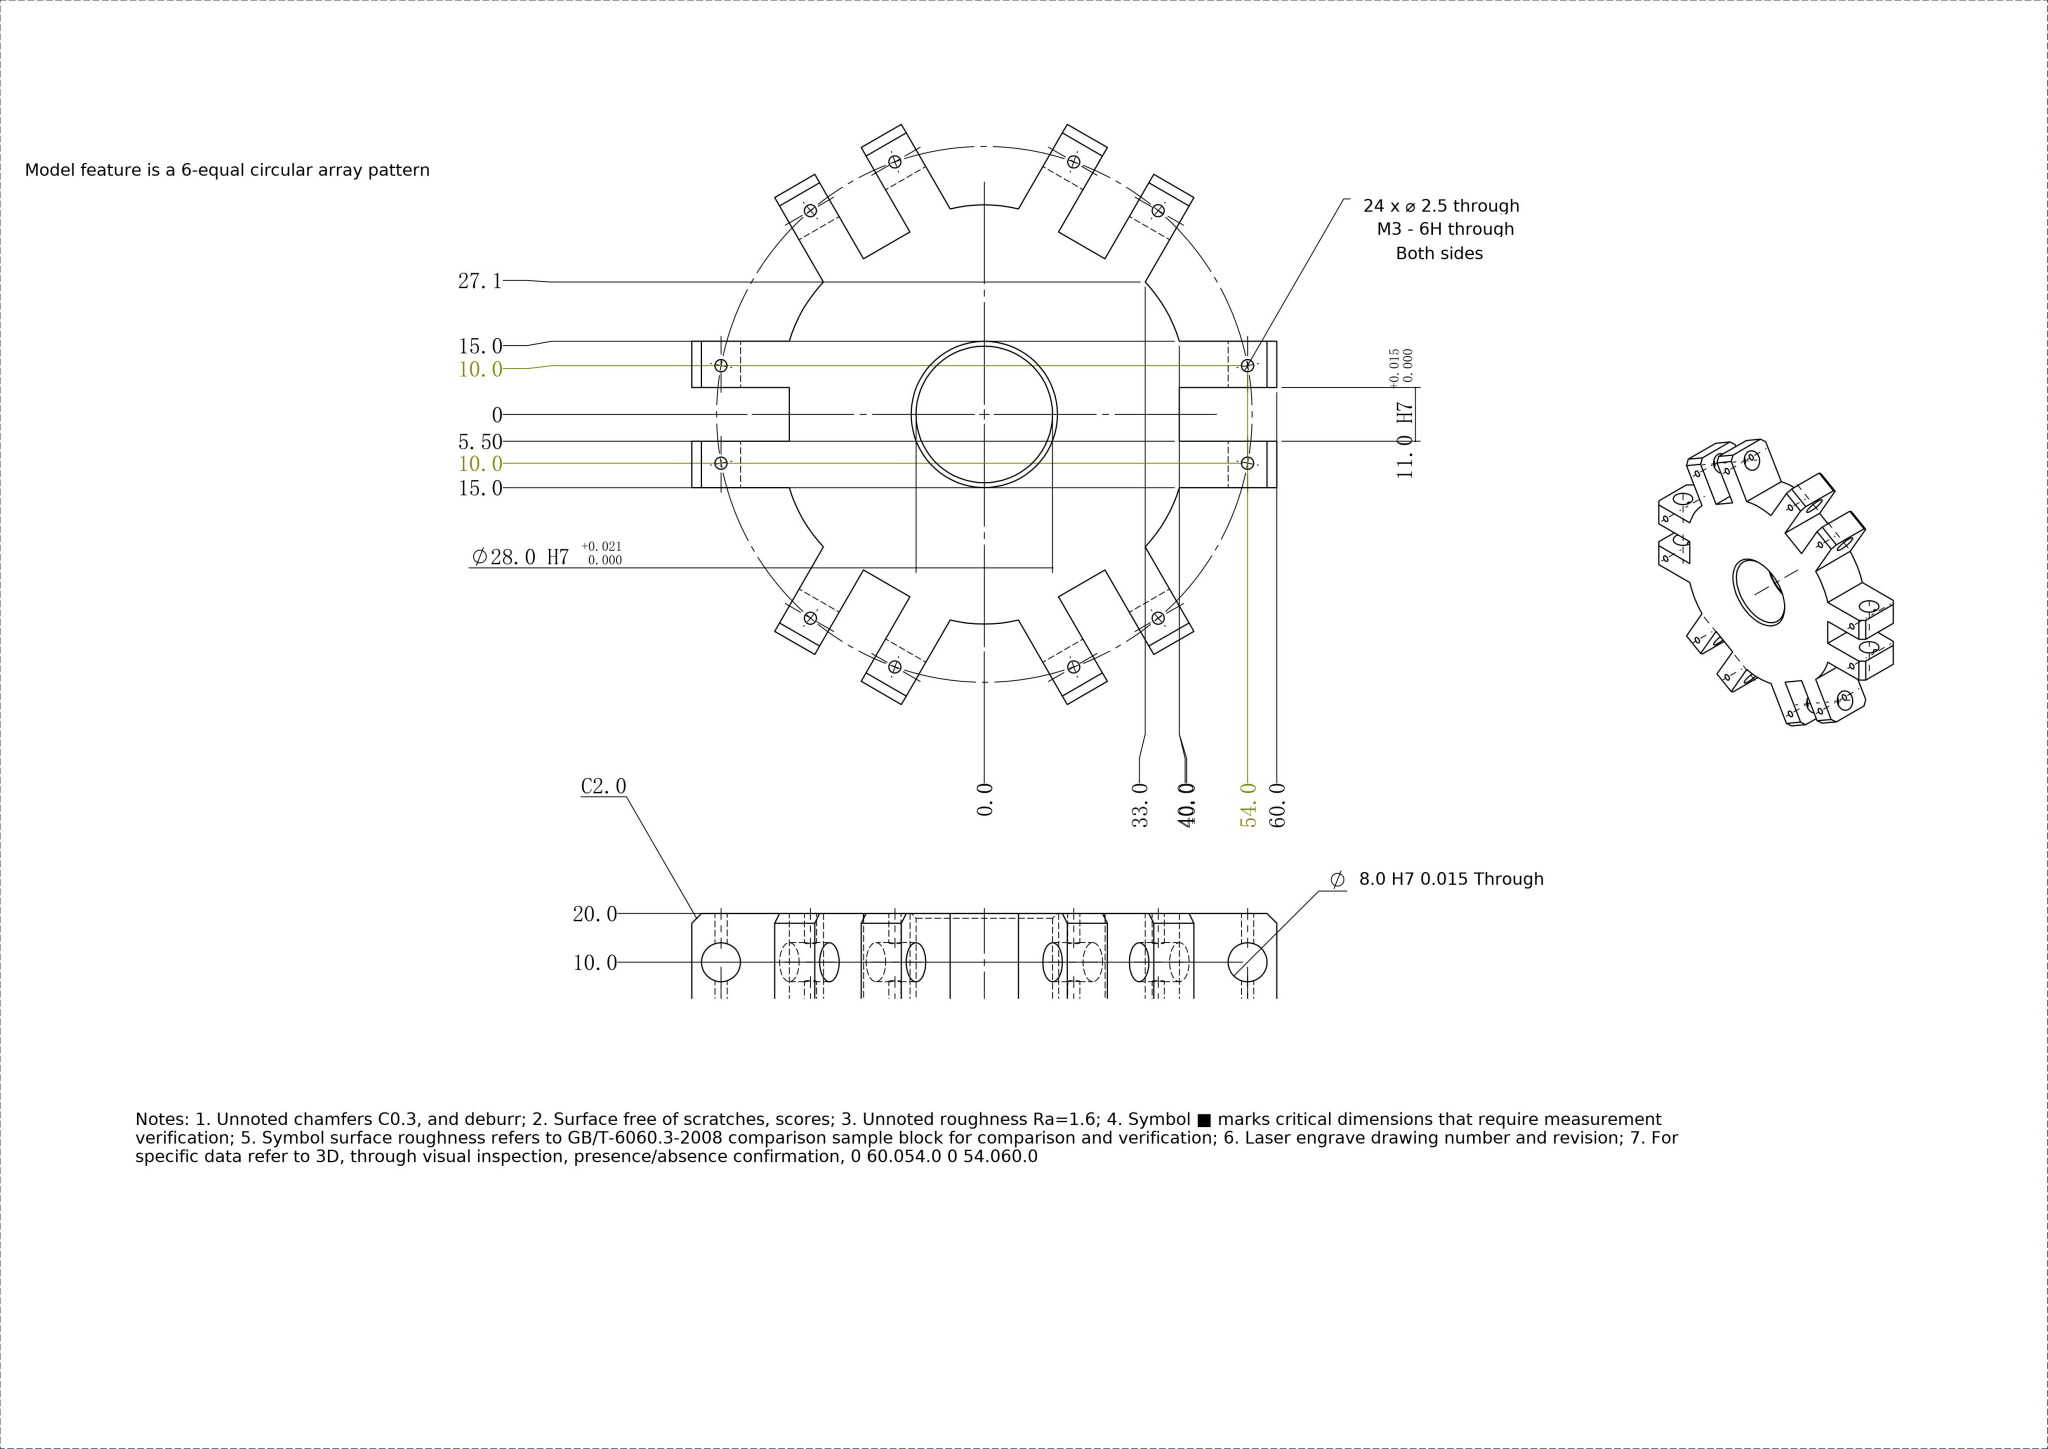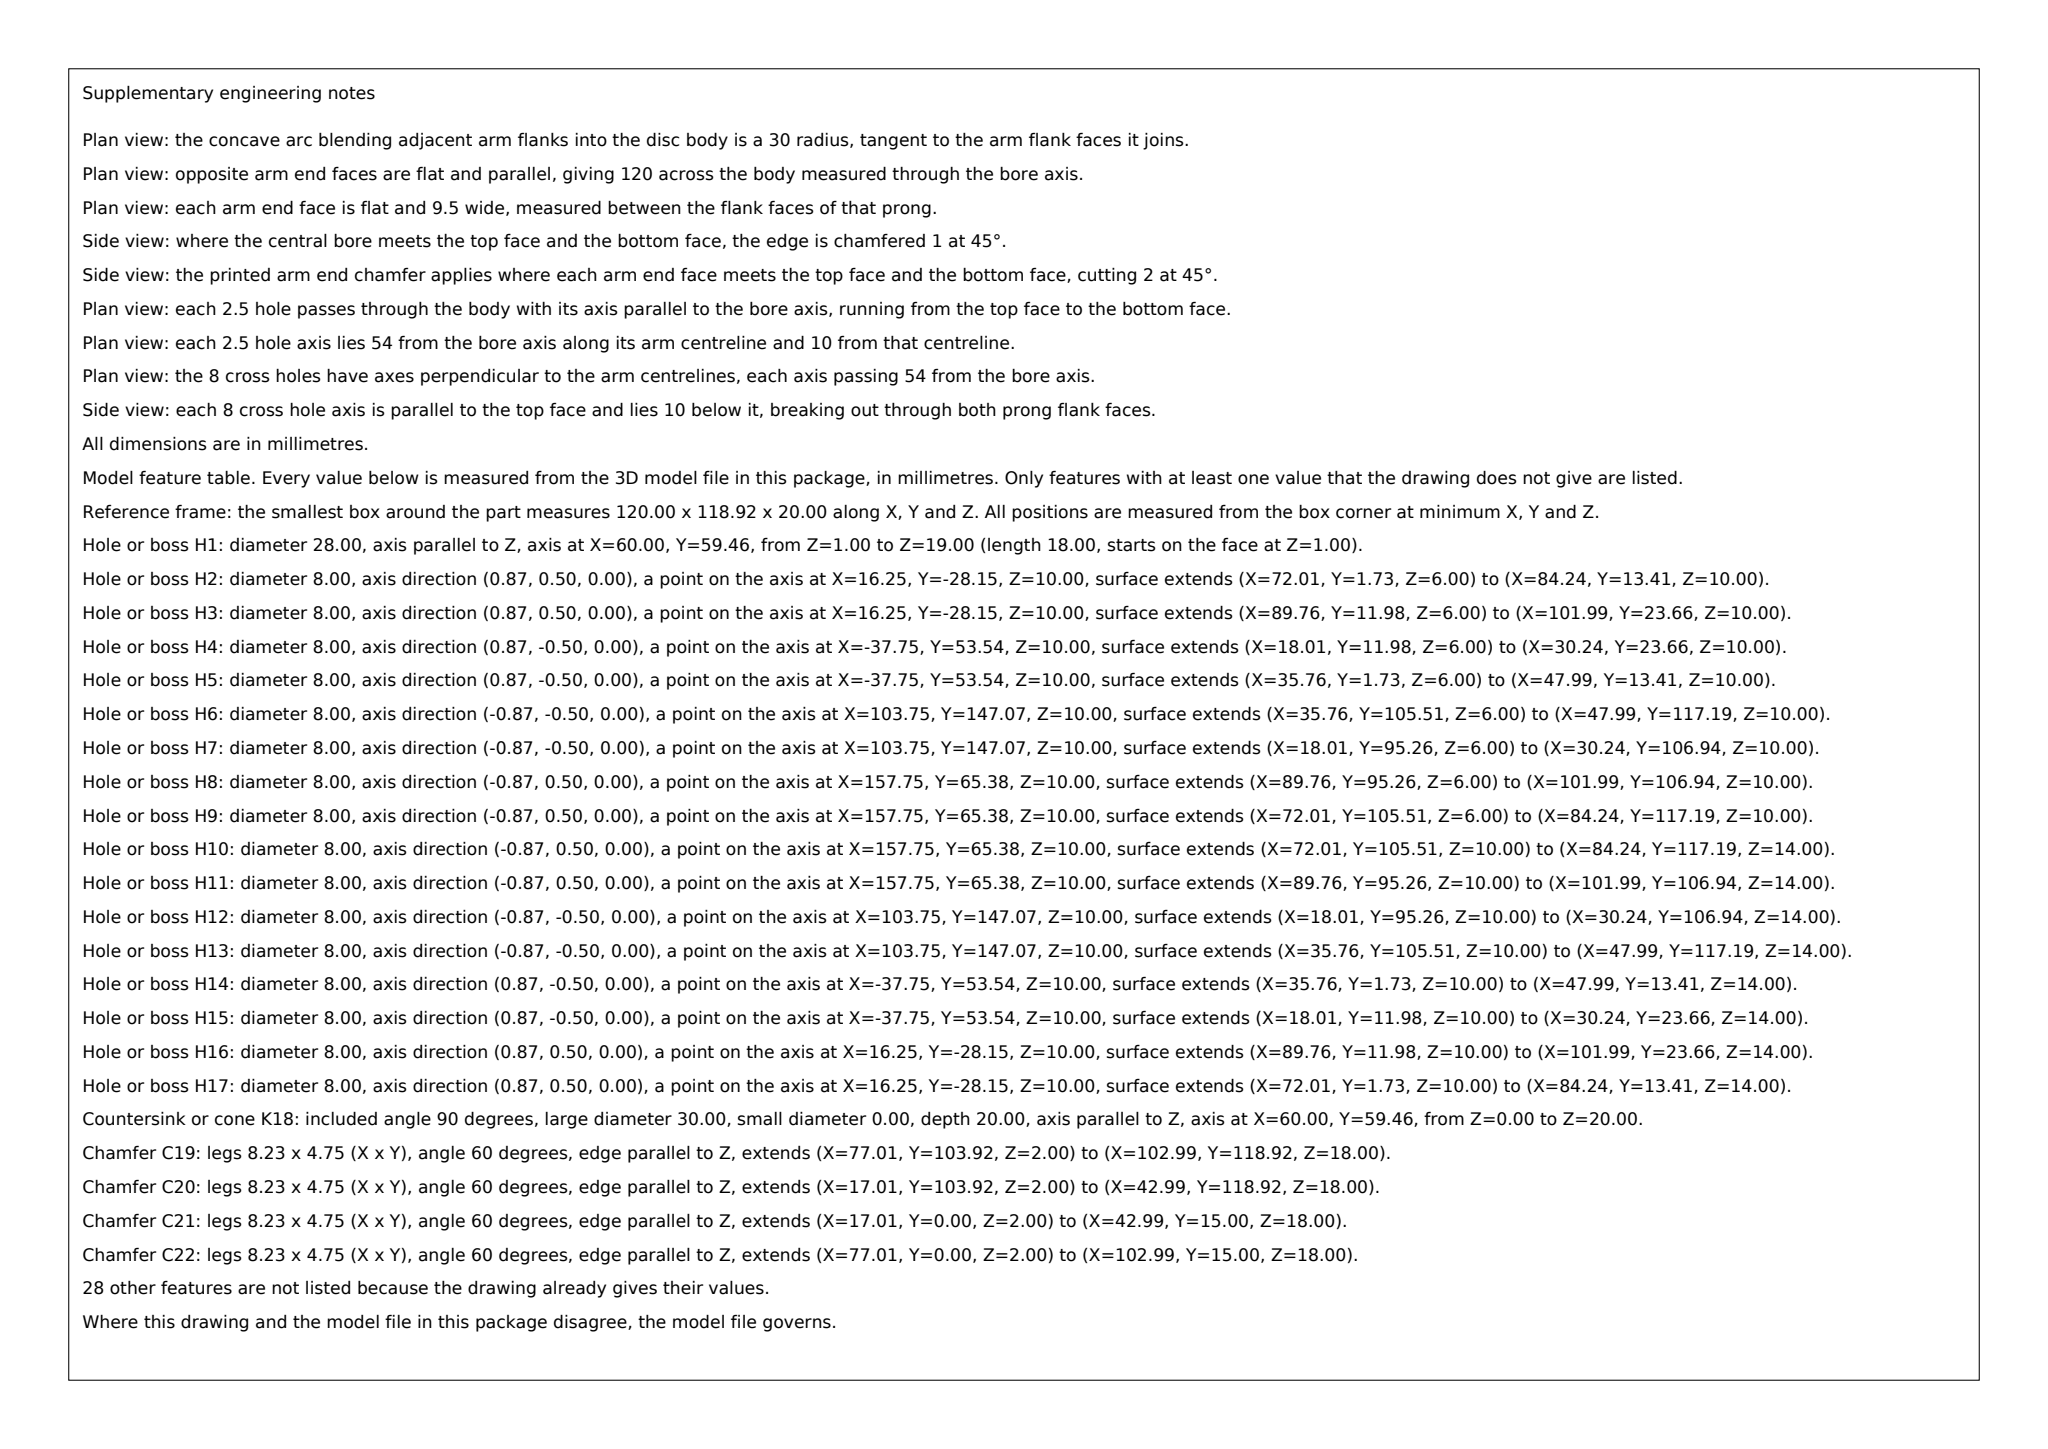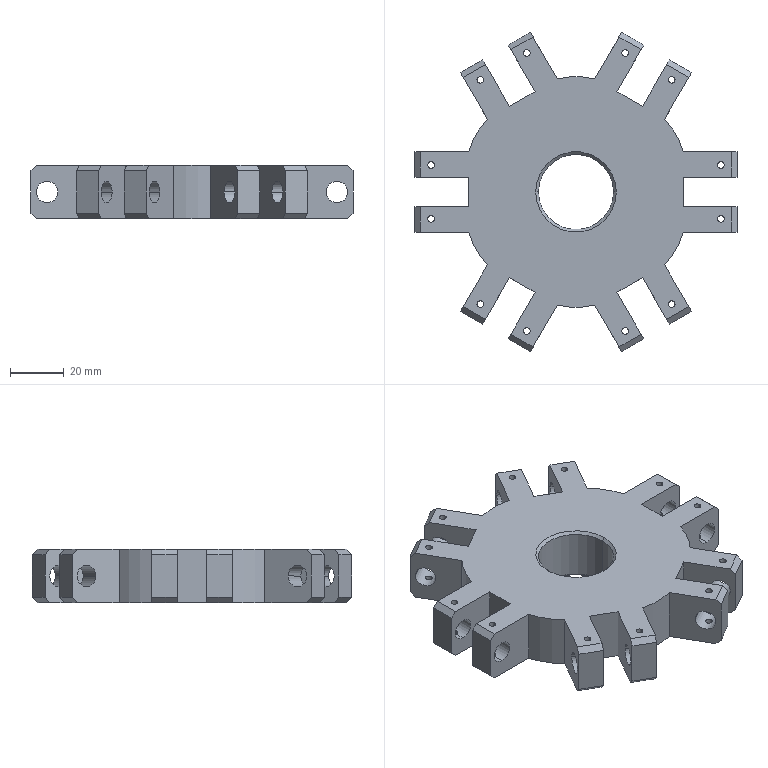Part | SolidWorks | mm | 1 solid | 152 faces | box 120 x 118.92 x 20 mm | volume 134677 mm3 | cylinder 80 | plane 68 | cone 4 | commonest cylinder face diameters 2.5 x48 8 x24 60 x6 28 x2
Drawing notes:
ALL DIMENSIONS IN MILLIMETRES (mm) UNLESS OTHERWISE STATED. | from the solid: STEP model facts header: units mm
OVERALL BODY ENVELOPE 120.0 MAX ACROSS OPPOSITE POCKET END FACES (X=0 TO X=120), 118.9 MAX ACROSS Y, ABOUT THE Ø28.0 H7 BORE AXIS. | from the solid: bbox_xyz [120.0, 118.923, 20.0]; axis_planes x=0.0 and x=120.0
OVERALL DISC THICKNESS 20.0, BOTH FACES FLAT AND PARALLEL (Z=0 AND Z=20). | from the solid: axis_planes z=0.0 and z=20.0, extent x[2.0,118.0] y[1.7,117.2]
6 INSERT POCKETS EQUALLY SPACED 60° ABOUT THE Ø28.0 H7 BORE AXIS; POCKET FLANK FACES INCLINED 30° TO X-AXIS / 60° TO Y-AXIS, RUNNING THROUGH THE FULL 20.0 THICKNESS. | from the solid: inclined_planes angle_to_xyz_axes [30.0,60.0,90.0], size [10.0,17.3,20.0], 16 off
EACH INSERT POCKET: 11.0 H7 SLOT, 20.0 DEEP FROM POCKET END FACE (X=120 TO X=100), THROUGH FULL 20.0 THICKNESS; JAW EACH SIDE 9.5 THICK, FACES 5.5 AND 15.0 FROM POCKET CENTRE LINE. | from the solid: axis_planes x=100.0 and x=20.0 extent y[54.0,65.0] z[0,20]; axis_planes y=44.5/54.0/65.0/74.5 at x[0,20] and x[100,120]
Ø8.0 H7 CROSS HOLE THRU BOTH JAWS, AXIS PERPENDICULAR TO POCKET SLOT, 6.0 FROM POCKET END FACE AND 10.0 FROM EACH DISC FACE (MID-THICKNESS); 1 PER POCKET, 6 PLACES. | from the solid: cylinders hole/bore 8.0 axis y at [114.0,-,10.0] from y 44.5 to 54.0 and 65.0 to 74.5 (and inclined equivalents)
24 x Ø2.5 THRU / M3-6H: 2 PER POCKET, AXES PARALLEL TO BORE AXIS, 10.0 EACH SIDE OF POCKET SLOT CENTRE LINE (20.0 APART) AND 6.0 FROM POCKET END FACE. | from the solid: cylinders hole/bore 2.5 axis z at [114.0,49.5] and [114.0,69.5] (part centre y=59.5), repeated 6x
6X R30.0 ARC CENTRES EQUALLY SPACED 60° ON A Ø26.0 BOLT CIRCLE ABOUT THE Ø28.0 H7 BORE AXIS. | from the solid: convex arc dia 60.0 axis z centres (48.8,53.0)(48.8,65.9)(60.0,46.5)(60.0,72.4)(71.2,53.0)(71.2,65.9) vs bore centre (60.0,59.5)
C2.0 x 45° CHAMFER ON EACH JAW END-FACE EDGE AT BOTH DISC FACES (Z=0 AND Z=20), 9.5 LONG ACROSS JAW - 4 PLACES PER POCKET, 24 PLACES TOTAL. | from the solid: inclined_planes angle_to_xyz_axes [45.0,90.0,45.0], size [2.0,9.5,2.0] at [0,44.5,0],[0,44.5,18],[0,65,0],[0,65,18],[118,...]